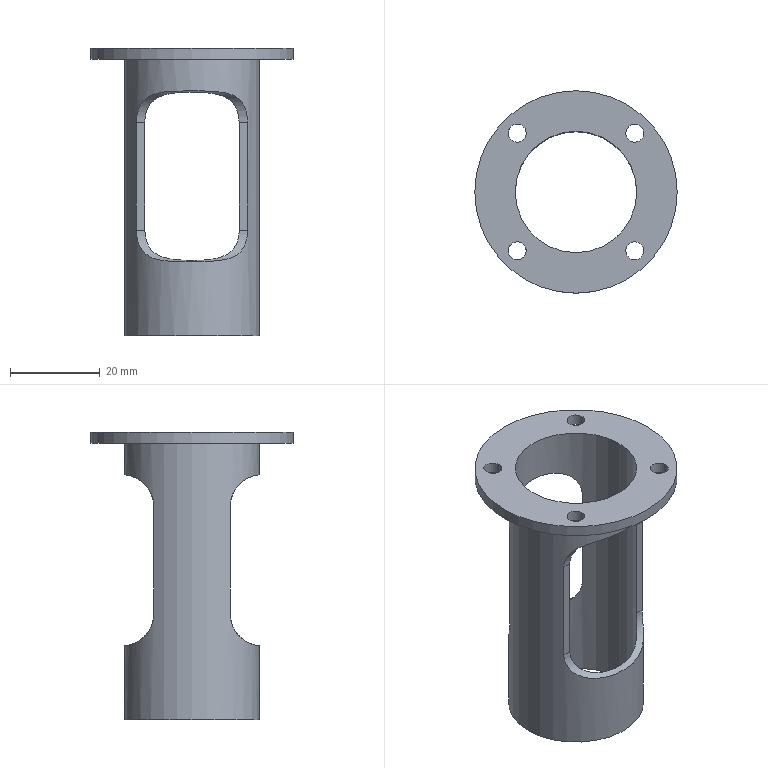Component | NX | LOWER_PISTON_CYLINDER | 1 solid | 18 faces | volume 7844 mm3 | cylinder 11 | plane 7 | commonest cylinder face diameters 14 x4 4 x4 30 x1 27 x1 45 x1